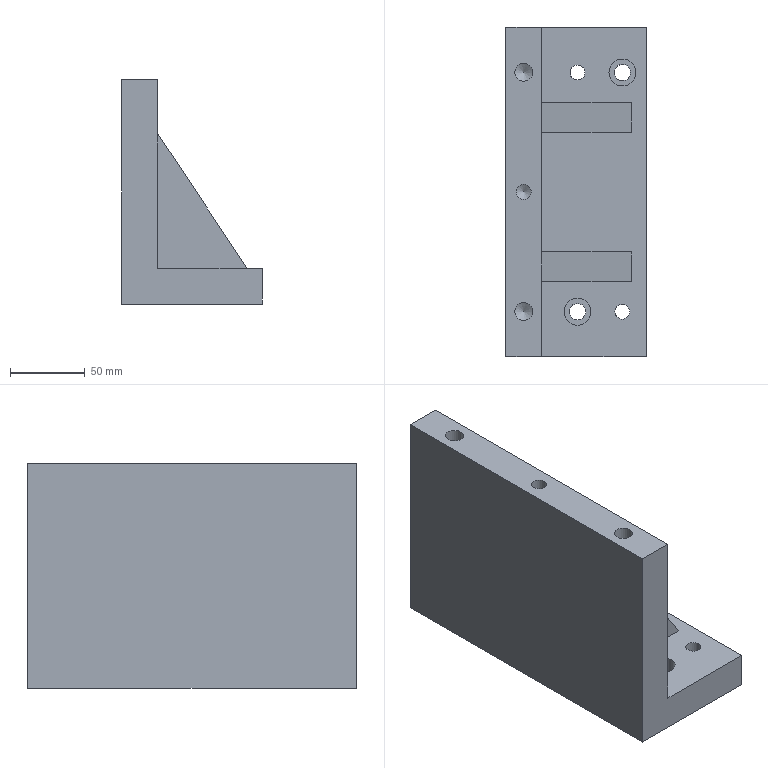Component | NX | ANGLE_IRON_2 | 1 solid | 28 faces | volume 1251380 mm3 | plane 16 | cylinder 9 | cone 3 | commonest cylinder face diameters 10 x3 11 x2 18 x2 12 x2